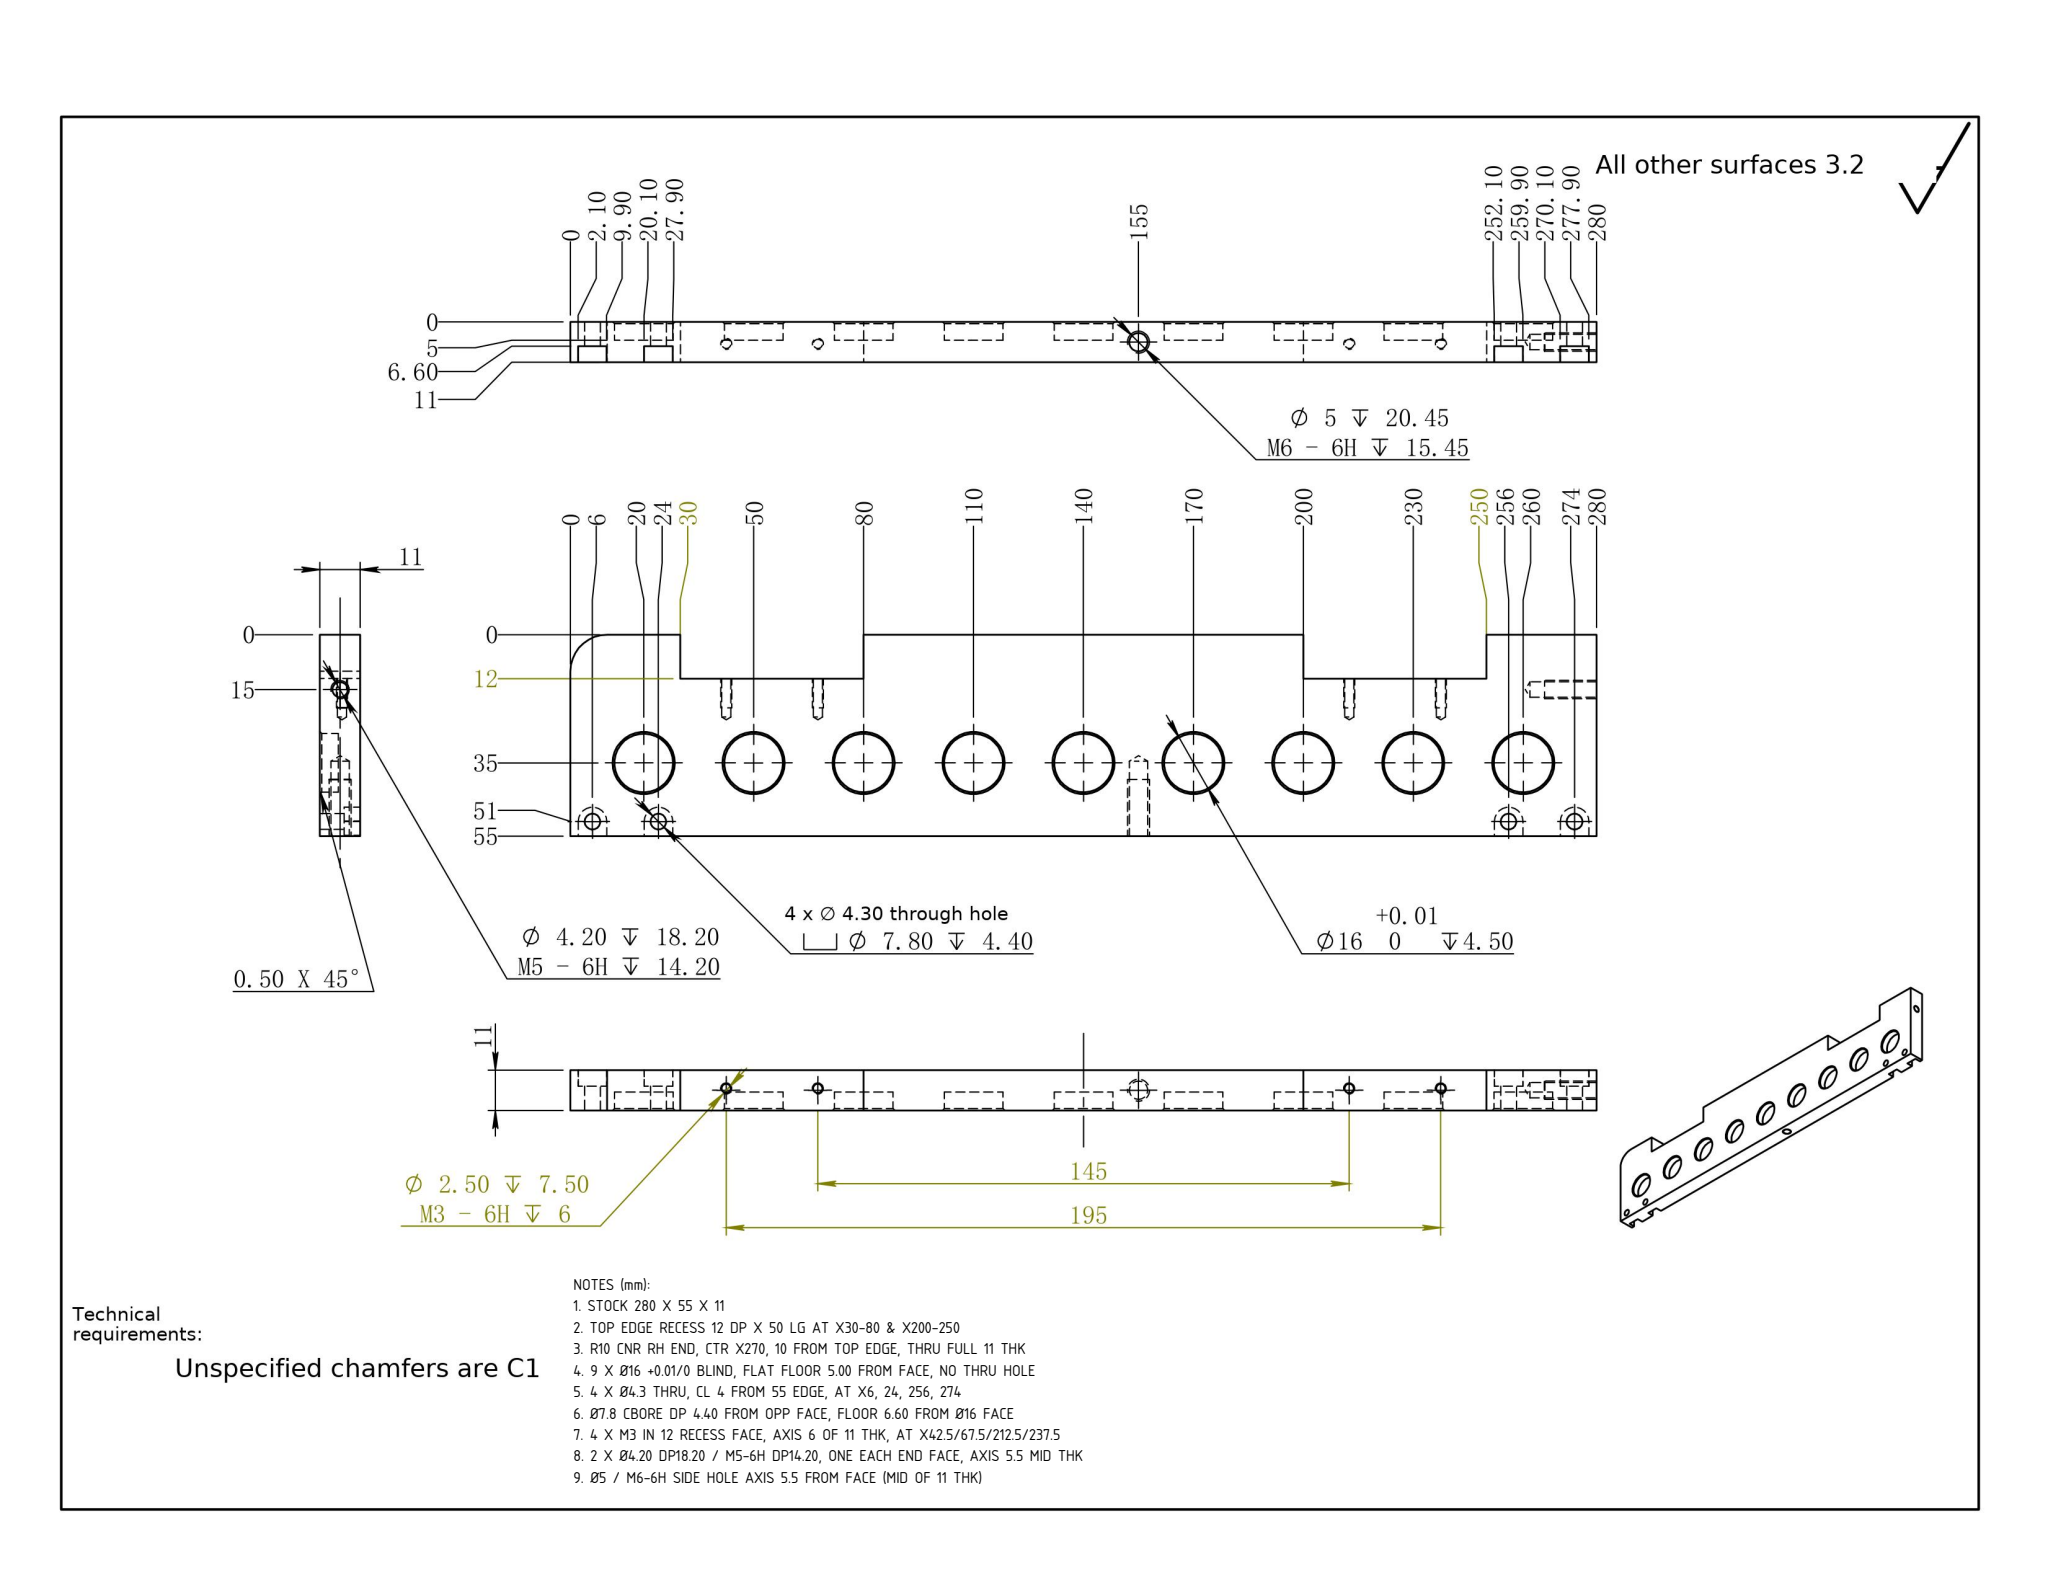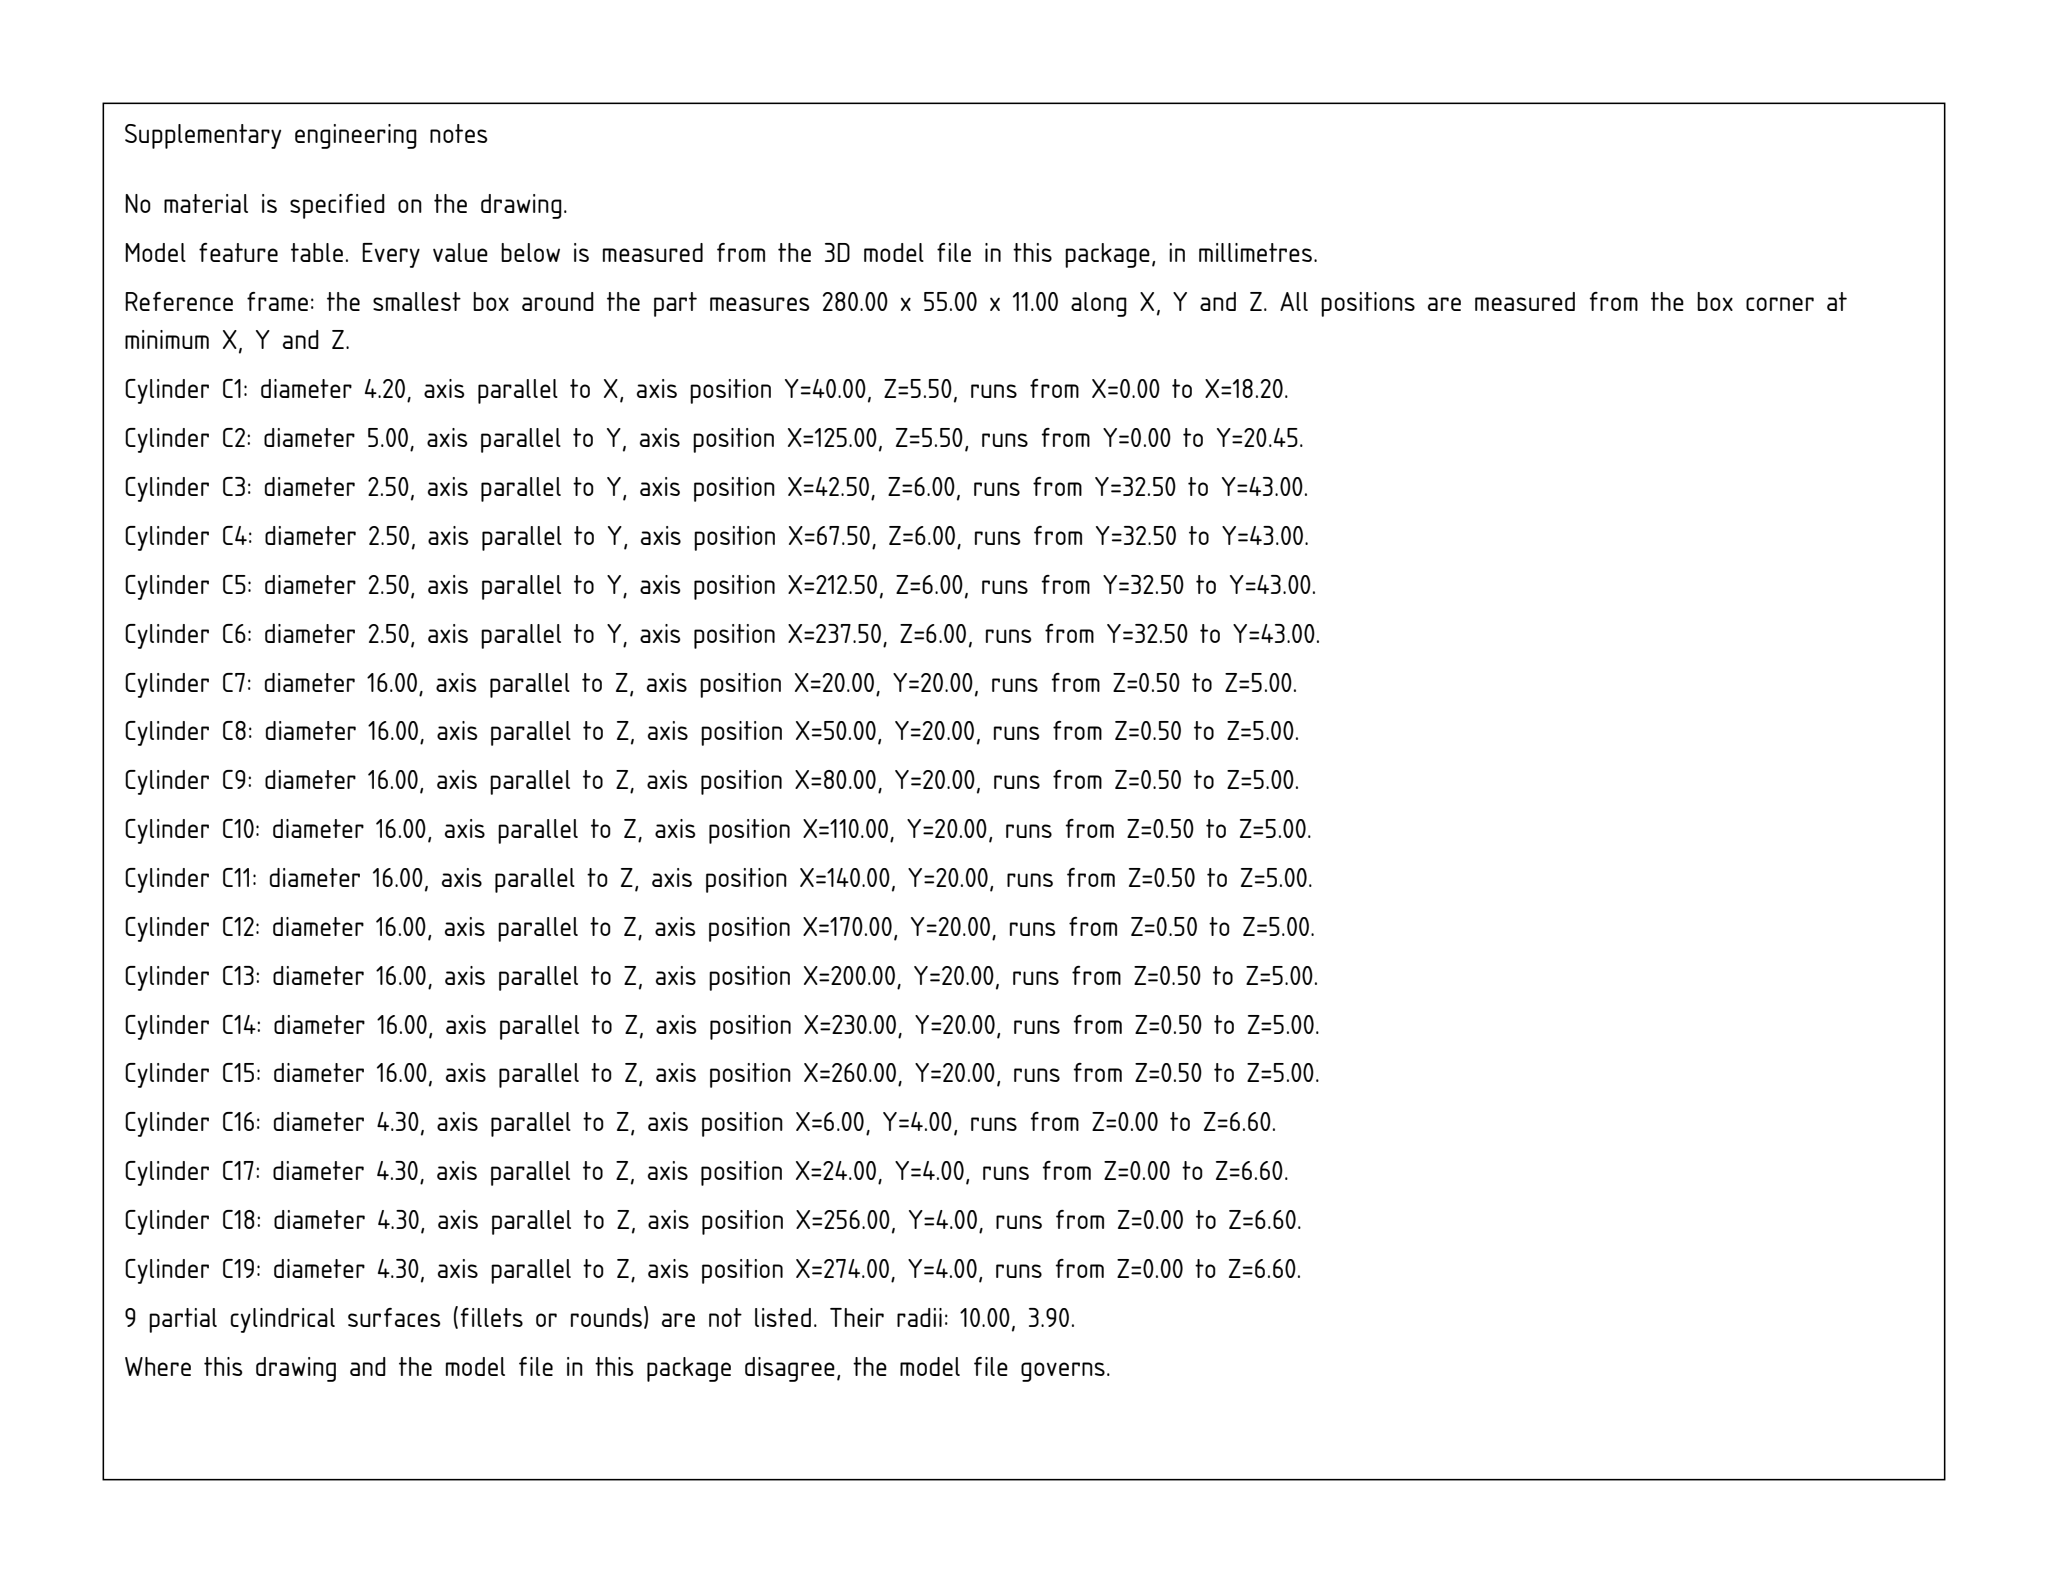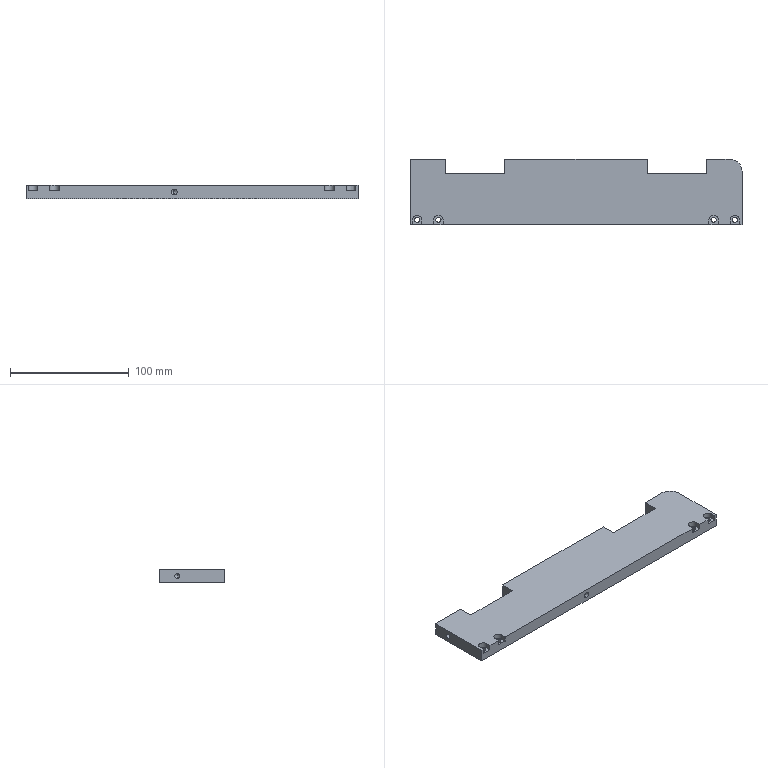Part | SolidWorks | mm | 1 solid | 116 faces | box 280 x 55 x 11 mm | volume 144625 mm3 | cylinder 51 | plane 35 | cone 30 | commonest cylinder face diameters 16 x18 7.8 x12 2.5 x8 4.3 x8 4.2 x2 5 x2 20 x1
Drawing notes:
STOCK 280 X 55 X 11 | from the solid: bbox_xyz [280.0, 55.0, 11.0]
TOP EDGE RECESS 12 DP X 50 LG AT X30-80 & X200-250 | from the solid: y=43.0 plane count 2 (55-12); x planes 30.0, 80.0, 200.0, 250.0
R10 CNR RH END, CTR X270, 10 FROM TOP EDGE, THRU FULL 11 THK | from the solid: cyl dia 20 axis z at (270,45) L11 = full thk; drawing Y = 55 - STEP Y = 10
9 X Ø16 +0.01/0 BLIND, FLAT FLOOR 5.00 FROM FACE, NO THRU HOLE | from the solid: Ø16 z-axis cyls L4.50 at x=20..260, y=20, 90° cone ref Ø17; z=5.0 plane count 9
4 X Ø4.3 THRU, CL 4 FROM 55 EDGE, AT X6, 24, 256, 274 | from the solid: Ø4.3 z-axis cyls at (6,4),(24,4),(256,4),(274,4), L6.6
Ø7.8 CBORE DP 4.40 FROM OPP FACE, FLOOR 6.60 FROM Ø16 FACE | from the solid: Ø7.8 z cyls L4.4 at same x,y as Ø4.3; z=6.6 plane count 4; 6.6+4.4=11 thk
4 X M3 IN 12 RECESS FACE, AXIS 6 OF 11 THK, AT X42.5/67.5/212.5/237.5 | from the solid: Ø2.5 y-axis cyls z=6.0 L10.5 from y=43 face; x=42.5, 67.5, 212.5, 237.5 (145 & 195)
2 X Ø4.20 DP18.20 / M5-6H DP14.20, ONE EACH END FACE, AXIS 5.5 MID THK | from the solid: [4.2,"x",[null,40.0,5.5],18.2,2]; 118° cone ref Ø4.2 count 2
Ø5 / M6-6H SIDE HOLE AXIS 5.5 FROM FACE (MID OF 11 THK) | from the solid: cyl dia 5.0 axis y, pos_other (x=125, z=5.5), L20.45
build123d program:
from build123d import *

# Parameters (mm, degrees)
SKETCH1_W                                       = 280
SKETCH1_H                                       = 55
BOSS_EXTRUDE1_DEPTH                             = 5.5
SKETCH2_R                                       = 8
CUT_EXTRUDE1_DEPTH                              = 5
LPATTERN1_COUNT                                 = 13
LPATTERN1_PITCH                                 = 30
M4_HEX_SOCKET_HEAD_CAP_SCREW_CBORE3_D           = 4.3
M4_HEX_SOCKET_HEAD_CAP_SCREW_CBORE3_CBORE_D     = 7.8
M4_HEX_SOCKET_HEAD_CAP_SCREW_CBORE3_CBORE_DEPTH = 4.4
CUT_EXTRUDE3_DEPTH                              = 143.828
FILLET1_R                                       = 10
M6_TAPPED_HOLE1_D                               = 5
M6_TAPPED_HOLE1_DEPTH                           = 20.45
M6_TAPPED_HOLE1_TIP                             = 1.502
M5_TAPPED_HOLE1_D                               = 4.2
M5_TAPPED_HOLE1_DEPTH                           = 18.2
M5_TAPPED_HOLE1_TIP                             = 1.262
CHAMFER1_SIZE                                   = 0.5
SKETCH13_W                                      = 50
SKETCH13_H                                      = 12
CUT_EXTRUDE4_DEPTH                              = 144.099
M3_TAPPED_HOLE1_AT_2_COUNT                      = 2
M3_TAPPED_HOLE1_AT_2_PITCH                      = 25


with BuildPart() as part:
    # Sketch1 → Boss-Extrude1 (new, symmetric)
    with BuildSketch(Plane.XY):
        Rectangle(SKETCH1_W, SKETCH1_H)
    extrude(amount=BOSS_EXTRUDE1_DEPTH, both=True)

    # Sketch2 → Cut-Extrude1 (cut)
    with BuildSketch(Plane.XY.offset(-5.5)):
        with Locations((120, -7.5)):
            Circle(SKETCH2_R)
    cut_extrude1 = extrude(amount=CUT_EXTRUDE1_DEPTH, mode=Mode.SUBTRACT)

    # LPattern1: Cut-Extrude1 ×13
    with Locations(*[(-i * LPATTERN1_PITCH, 0, 0) for i in range(1, LPATTERN1_COUNT)]):
        add(cut_extrude1, mode=Mode.SUBTRACT)

    # M4 Hex Socket Head Cap Screw CBORE3 (through all)
    with Locations(Plane(origin=(0, 0, 5.5), x_dir=(-1, 0, 0), z_dir=(0, 0, 1))):
        with Locations((116, 23.5), (134, 23.5), (-134, 23.5), (-116, 23.5)):
            CounterBoreHole(M4_HEX_SOCKET_HEAD_CAP_SCREW_CBORE3_D / 2, M4_HEX_SOCKET_HEAD_CAP_SCREW_CBORE3_CBORE_D / 2, M4_HEX_SOCKET_HEAD_CAP_SCREW_CBORE3_CBORE_DEPTH)

    # Sketch8 → Cut-Extrude3 (cut, through all)
    with BuildSketch(Plane.XY.offset(1.1)):
        with BuildLine():
            Line((-112.1, -23.5), (-112.1, -27.4))
            ThreePointArc((-112.1, -27.4), (-116, -31.3), (-119.9, -27.4))
            Line((-119.9, -27.4), (-119.9, -23.5))
            ThreePointArc((-119.9, -23.5), (-116, -19.6), (-112.1, -23.5))
        make_face()
        with BuildLine():
            Line((-130.1, -23.5), (-130.1, -27.4))
            ThreePointArc((-130.1, -27.4), (-134, -31.3), (-137.9, -27.4))
            Line((-137.9, -27.4), (-137.9, -23.5))
            ThreePointArc((-137.9, -23.5), (-134, -19.6), (-130.1, -23.5))
        make_face()
        with BuildLine():
            Line((137.9, -23.5), (137.9, -27.4))
            ThreePointArc((137.9, -27.4), (134, -31.3), (130.1, -27.4))
            Line((130.1, -27.4), (130.1, -23.5))
            ThreePointArc((130.1, -23.5), (134, -19.6), (137.9, -23.5))
        make_face()
        with BuildLine():
            Line((119.9, -23.5), (119.9, -27.4))
            ThreePointArc((119.9, -27.4), (116, -31.3), (112.1, -27.4))
            Line((112.1, -27.4), (112.1, -23.5))
            ThreePointArc((112.1, -23.5), (116, -19.6), (119.9, -23.5))
        make_face()
    extrude(amount=CUT_EXTRUDE3_DEPTH, mode=Mode.SUBTRACT)

    # Fillet1
    fillet1_edges = [part.edges().sort_by_distance(p)[0] for p in [
        (140, 27.5, 0),
    ]]
    fillet(fillet1_edges, radius=FILLET1_R)

    # M6 Tapped Hole1
    with Locations(Plane(origin=(0, -27.5, 0), x_dir=(-1, 0, 0), z_dir=(0, -1, 0))):
        with Locations((15, 0)):
            Hole(M6_TAPPED_HOLE1_D / 2, depth=M6_TAPPED_HOLE1_DEPTH)
            with Locations((0, 0, -(M6_TAPPED_HOLE1_DEPTH + M6_TAPPED_HOLE1_TIP / 2))):  # 118° drill point
                Cone(0, M6_TAPPED_HOLE1_D / 2, M6_TAPPED_HOLE1_TIP, mode=Mode.SUBTRACT)

    # M5 Tapped Hole1
    with Locations(Plane.ZY.offset(140)):
        with Locations((0, 12.5)):
            Hole(M5_TAPPED_HOLE1_D / 2, depth=M5_TAPPED_HOLE1_DEPTH)
            with Locations((0, 0, -(M5_TAPPED_HOLE1_DEPTH + M5_TAPPED_HOLE1_TIP / 2))):  # 118° drill point
                Cone(0, M5_TAPPED_HOLE1_D / 2, M5_TAPPED_HOLE1_TIP, mode=Mode.SUBTRACT)

    # Chamfer1
    chamfer1_edges = [part.edges().sort_by_distance(p)[0] for p in [
        (112, -7.5, -5.5),
        (82, -7.5, -5.5),
        (52, -7.5, -5.5),
        (22, -7.5, -5.5),
        (-8, -7.5, -5.5),
        (-38, -7.5, -5.5),
        (-68, -7.5, -5.5),
        (-98, -7.5, -5.5),
        (-128, -7.5, -5.5),
    ]]
    chamfer(chamfer1_edges, length=CHAMFER1_SIZE)

    # Sketch13 → Cut-Extrude4 (cut, through all)
    with BuildSketch(Plane.XY.offset(5.5)):
        with Locations((85, 21.5)):
            Rectangle(SKETCH13_W, SKETCH13_H)
    cut_extrude4 = extrude(amount=-CUT_EXTRUDE4_DEPTH, mode=Mode.SUBTRACT)

    # Mirror1: Cut-Extrude4 across plane
    add(cut_extrude4.mirror(Plane(origin=(0, 0, 0), x_dir=(0, 0, 1), z_dir=(1, 0, 0))), mode=Mode.SUBTRACT)

    # Sketch15 → M3 Tapped Hole1 (revolve, cut)
    with BuildSketch(Plane(origin=(72.5, 15.5, 0.5), x_dir=(0, 0, 1), z_dir=(1, 0, 0))):
        Polygon((0, 0), (0, 11.251), (1.25, 10.5), (1.25, 0), align=None)
    m3_tapped_hole1 = revolve(axis=Axis((72.5, 21.85, 0.5), (0, -1, 0)), mode=Mode.SUBTRACT)

    # M3 Tapped Hole1 at 2: M3 Tapped Hole1 ×2
    with Locations(*[(i * M3_TAPPED_HOLE1_AT_2_PITCH, 0, 0) for i in range(1, M3_TAPPED_HOLE1_AT_2_COUNT)]):
        add(m3_tapped_hole1, mode=Mode.SUBTRACT)

    # Mirror2: M3 Tapped Hole1 across plane
    add(m3_tapped_hole1.mirror(Plane(origin=(0, 0, 0), x_dir=(0, 0, 1), z_dir=(1, 0, 0))), mode=Mode.SUBTRACT)

    # Mirror2 copy 1 sketch → Mirror2 copy 1 (revolve, cut)
    with BuildSketch(Plane(origin=(-97.5, 15.5, 0.5), x_dir=(0, 0, 1), z_dir=(-1, 0, 0))):
        Polygon((0, 0), (0, -11.251), (1.25, -10.5), (1.25, 0), align=None)
    revolve(axis=Axis((-97.5, 21.85, 0.5), (0, 1, 0)), mode=Mode.SUBTRACT)


solid = part.part